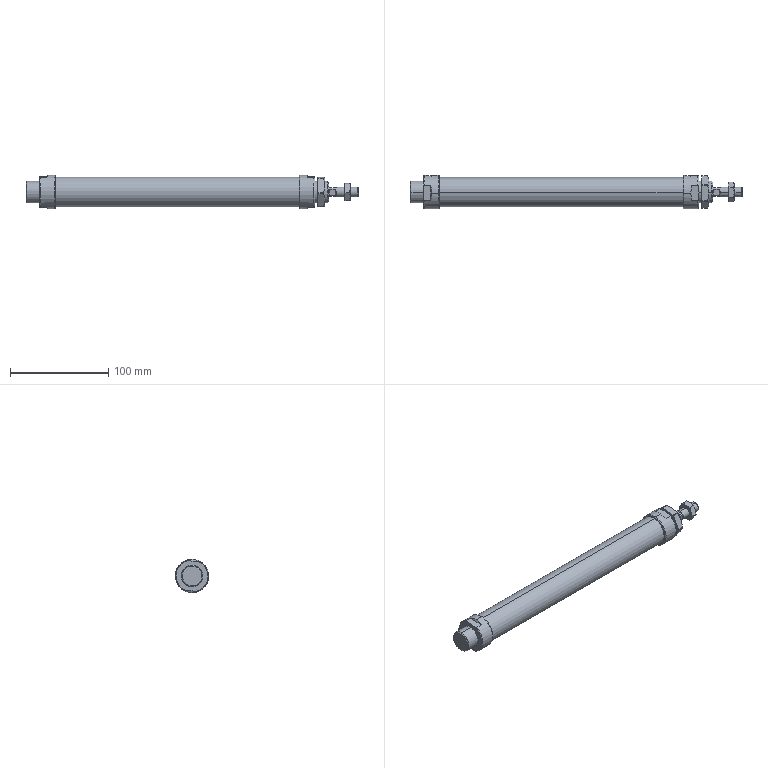Component | SolidWorks | AluminumAlloyMiniCylinder-MAL-25x210-S-CM-AIRTAC-1 | 4 solids | 149 faces | volume 130882 mm3 | plane 53 | cylinder 40 | cone 40 | torus 16 | commonest cylinder face diameters 10 x6 22 x6 33 x6 24.5 x6 8.566 x4 34 x4 25 x2 30 x2 | material Q235A